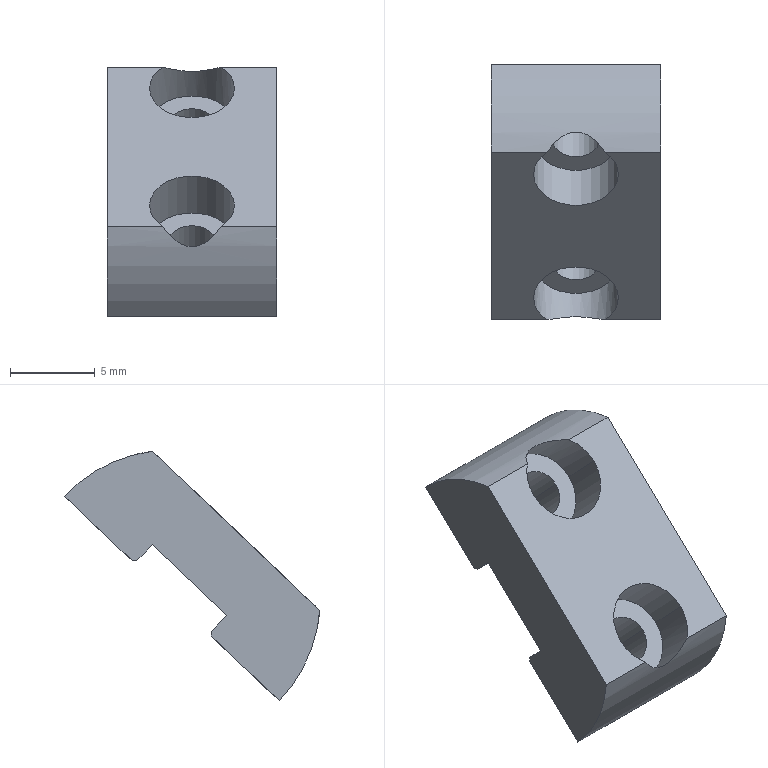Component | SolidWorks | JJDJR-3060-E-006-1 | 1 solid | 22 faces | box 10 x 15.06 x 14.71 mm | volume 656 mm3 | plane 12 | cylinder 10 | commonest cylinder face diameters 2.8 x4 5 x4 17.5 x2 | material 40Cr
build123d program:
from build123d import *

# Parameters (mm, degrees)
BOSS_EXTRUDE1_DEPTH                               = 5
M2_5_HEX_SOCKET_HEAD_CAP_SCREW_CBORE2_D           = 2.8
M2_5_HEX_SOCKET_HEAD_CAP_SCREW_CBORE2_CBORE_D     = 5
M2_5_HEX_SOCKET_HEAD_CAP_SCREW_CBORE2_CBORE_DEPTH = 6.5
CUT_EXTRUDE1_DEPTH                                = 16.91
CUT_EXTRUDE1_DEPTH_BACK                           = 16.91
CHAMFER1_SIZE                                     = 0.2


with BuildPart() as part:
    # Sketch1 → Boss-Extrude1 (new, symmetric)
    with BuildSketch(Plane.XY):
        with BuildLine():
            Line((-3.025, 0), (-8.75, 0))
            ThreePointArc((-8.75, 0), (0, 8.75), (8.75, 0))
            Line((8.75, 0), (3.025, 0))
            Line((3.025, 0), (3.025, 1.5))
            Line((3.025, 1.5), (-3.025, 1.5))
            Line((-3.025, 1.5), (-3.025, 0))
        make_face()
    extrude(amount=BOSS_EXTRUDE1_DEPTH, both=True)

    # M2.5 Hex Socket Head Cap Screw CBORE2 (through all)
    with Locations(Plane(origin=(0, 9, 0), x_dir=(1, 0, 0), z_dir=(0, 1, 0))):
        with Locations((5, 0), (-5, 0)):
            CounterBoreHole(M2_5_HEX_SOCKET_HEAD_CAP_SCREW_CBORE2_D / 2, M2_5_HEX_SOCKET_HEAD_CAP_SCREW_CBORE2_CBORE_D / 2, M2_5_HEX_SOCKET_HEAD_CAP_SCREW_CBORE2_CBORE_DEPTH)

    # Sketch4 → Cut-Extrude1 (cut, two sides: drawn at the far end of the back side and taken through both)
    with BuildSketch(Plane.XY.offset(5).offset(-CUT_EXTRUDE1_DEPTH_BACK)):
        Polygon((-57.338, 5.5), (-9.087, 5.5), (9.567, 5.5), (57.818, 5.5), (57.818, 102.002), (-57.338, 102.002), align=None)
    extrude(amount=CUT_EXTRUDE1_DEPTH + CUT_EXTRUDE1_DEPTH_BACK, mode=Mode.SUBTRACT)

    # Chamfer1
    chamfer1_edges = [part.edges().sort_by_distance(p)[0] for p in [
        (-3.025, 0, 0),
        (3.025, 0, 0),
    ]]
    chamfer(chamfer1_edges, length=CHAMFER1_SIZE)


solid = part.part

# Placed as in the assembly
solid = solid.moved(Location((-123.59, -29.263, -16.52), (133.57, 90, 0)))
STEP:
#1=COLOUR_RGB('',0.7922,0.8196,0.9333);
#2=FILL_AREA_STYLE_COLOUR('',#1);
#3=FILL_AREA_STYLE('',(#2));
#4=SURFACE_STYLE_FILL_AREA(#3);
#5=SURFACE_SIDE_STYLE('',(#4));
#6=SURFACE_STYLE_USAGE(.BOTH.,#5);
#7=PRESENTATION_STYLE_ASSIGNMENT((#6));
#8=CARTESIAN_POINT('',(-4.921,-1.009,-0.5147));
#9=VERTEX_POINT('',#8);
#10=CARTESIAN_POINT('',(-4.811,-1.009,-0.5147));
#11=VERTEX_POINT('',#10);
#12=CARTESIAN_POINT('',(-4.866,-1.009,-0.5147));
#13=DIRECTION('',(0.,-0.6892,0.7245));
#14=DIRECTION('',(1.,0.,0.));
#15=AXIS2_PLACEMENT_3D('',#12,#13,#14);
#16=CIRCLE('',#15,0.05512);
#17=EDGE_CURVE('',#9,#11,#16,.T.);
#18=ORIENTED_EDGE('',*,*,#17,.F.);
#19=CARTESIAN_POINT('',(-4.921,-1.077,-0.4434));
#20=VERTEX_POINT('',#19);
#21=CARTESIAN_POINT('',(-4.921,-1.254,-0.258));
#22=DIRECTION('',(0.,-0.6892,0.7245));
#23=VECTOR('',#22,39.37);
#24=LINE('',#21,#23);
#25=EDGE_CURVE('',#9,#20,#24,.T.);
#26=ORIENTED_EDGE('',*,*,#25,.T.);
#27=CARTESIAN_POINT('',(-4.811,-1.077,-0.4434));
#28=VERTEX_POINT('',#27);
#29=CARTESIAN_POINT('',(-4.866,-1.077,-0.4434));
#30=DIRECTION('',(0.,-0.6892,0.7245));
#31=DIRECTION('',(1.,0.,0.));
#32=AXIS2_PLACEMENT_3D('',#29,#30,#31);
#33=CIRCLE('',#32,0.05512);
#34=EDGE_CURVE('',#20,#28,#33,.T.);
#35=ORIENTED_EDGE('',*,*,#34,.T.);
#36=CARTESIAN_POINT('',(-4.811,-1.254,-0.258));
#37=DIRECTION('',(0.,-0.6892,0.7245));
#38=VECTOR('',#37,39.37);
#39=LINE('',#36,#38);
#40=EDGE_CURVE('',#11,#28,#39,.T.);
#41=ORIENTED_EDGE('',*,*,#40,.F.);
#42=EDGE_LOOP('',(#18,#26,#35,#41));
#43=FACE_OUTER_BOUND('',#42,.T.);
#44=CARTESIAN_POINT('',(-4.866,-1.254,-0.258));
#45=DIRECTION('',(0.,-0.6892,0.7245));
#46=DIRECTION('',(1.,0.,0.));
#47=AXIS2_PLACEMENT_3D('',#44,#45,#46);
#48=CYLINDRICAL_SURFACE('',#47,0.05512);
#49=ADVANCED_FACE('',(#43),#48,.F.);
#50=CARTESIAN_POINT('',(-4.921,-1.295,-0.7861));
#51=VERTEX_POINT('',#50);
#52=CARTESIAN_POINT('',(-4.811,-1.295,-0.7861));
#53=VERTEX_POINT('',#52);
#54=CARTESIAN_POINT('',(-4.866,-1.295,-0.7861));
#55=DIRECTION('',(0.,-0.6892,0.7245));
#56=DIRECTION('',(1.,0.,0.));
#57=AXIS2_PLACEMENT_3D('',#54,#55,#56);
#58=CIRCLE('',#57,0.05512);
#59=EDGE_CURVE('',#51,#53,#58,.T.);
#60=ORIENTED_EDGE('',*,*,#59,.F.);
#61=CARTESIAN_POINT('',(-4.921,-1.363,-0.7148));
#62=VERTEX_POINT('',#61);
#63=CARTESIAN_POINT('',(-4.921,-1.539,-0.5294));
#64=DIRECTION('',(0.,-0.6892,0.7245));
#65=VECTOR('',#64,39.37);
#66=LINE('',#63,#65);
#67=EDGE_CURVE('',#51,#62,#66,.T.);
#68=ORIENTED_EDGE('',*,*,#67,.T.);
#69=CARTESIAN_POINT('',(-4.811,-1.363,-0.7148));
#70=VERTEX_POINT('',#69);
#71=CARTESIAN_POINT('',(-4.866,-1.363,-0.7148));
#72=DIRECTION('',(0.,-0.6892,0.7245));
#73=DIRECTION('',(1.,0.,0.));
#74=AXIS2_PLACEMENT_3D('',#71,#72,#73);
#75=CIRCLE('',#74,0.05512);
#76=EDGE_CURVE('',#62,#70,#75,.T.);
#77=ORIENTED_EDGE('',*,*,#76,.T.);
#78=CARTESIAN_POINT('',(-4.811,-1.539,-0.5294));
#79=DIRECTION('',(0.,-0.6892,0.7245));
#80=VECTOR('',#79,39.37);
#81=LINE('',#78,#80);
#82=EDGE_CURVE('',#53,#70,#81,.T.);
#83=ORIENTED_EDGE('',*,*,#82,.F.);
#84=EDGE_LOOP('',(#60,#68,#77,#83));
#85=FACE_OUTER_BOUND('',#84,.T.);
#86=CARTESIAN_POINT('',(-4.866,-1.539,-0.5294));
#87=DIRECTION('',(0.,-0.6892,0.7245));
#88=DIRECTION('',(1.,0.,0.));
#89=AXIS2_PLACEMENT_3D('',#86,#87,#88);
#90=CYLINDRICAL_SURFACE('',#89,0.05512);
#91=ADVANCED_FACE('',(#85),#90,.F.);
#92=CARTESIAN_POINT('',(-4.964,-1.077,-0.4434));
#93=VERTEX_POINT('',#92);
#94=CARTESIAN_POINT('',(-4.767,-1.077,-0.4434));
#95=VERTEX_POINT('',#94);
#96=CARTESIAN_POINT('',(-4.866,-1.077,-0.4434));
#97=DIRECTION('',(0.,-0.6892,0.7245));
#98=DIRECTION('',(1.,0.,0.));
#99=AXIS2_PLACEMENT_3D('',#96,#97,#98);
#100=CIRCLE('',#99,0.09843);
#101=EDGE_CURVE('',#93,#95,#100,.T.);
#102=ORIENTED_EDGE('',*,*,#101,.F.);
#103=CARTESIAN_POINT('',(-4.964,-1.159,-0.3578));
#104=VERTEX_POINT('',#103);
#105=CARTESIAN_POINT('',(-4.964,-1.254,-0.258));
#106=DIRECTION('',(0.,-0.6892,0.7245));
#107=VECTOR('',#106,39.37);
#108=LINE('',#105,#107);
#109=EDGE_CURVE('',#93,#104,#108,.T.);
#110=ORIENTED_EDGE('',*,*,#109,.T.);
#111=CARTESIAN_POINT('',(-4.767,-1.159,-0.3578));
#112=VERTEX_POINT('',#111);
#113=CARTESIAN_POINT('',(-4.866,-1.159,-0.3578));
#114=DIRECTION('',(-0.,0.6892,-0.7245));
#115=DIRECTION('',(1.,0.,0.));
#116=AXIS2_PLACEMENT_3D('',#113,#114,#115);
#117=CIRCLE('',#116,0.09843);
#118=EDGE_CURVE('',#112,#104,#117,.T.);
#119=ORIENTED_EDGE('',*,*,#118,.F.);
#120=CARTESIAN_POINT('',(-4.767,-1.254,-0.258));
#121=DIRECTION('',(0.,-0.6892,0.7245));
#122=VECTOR('',#121,39.37);
#123=LINE('',#120,#122);
#124=EDGE_CURVE('',#95,#112,#123,.T.);
#125=ORIENTED_EDGE('',*,*,#124,.F.);
#126=EDGE_LOOP('',(#102,#110,#119,#125));
#127=FACE_OUTER_BOUND('',#126,.T.);
#128=CARTESIAN_POINT('',(-4.866,-1.254,-0.258));
#129=DIRECTION('',(0.,-0.6892,0.7245));
#130=DIRECTION('',(1.,0.,0.));
#131=AXIS2_PLACEMENT_3D('',#128,#129,#130);
#132=CYLINDRICAL_SURFACE('',#131,0.09843);
#133=ADVANCED_FACE('',(#127),#132,.F.);
#134=CARTESIAN_POINT('',(-4.964,-1.363,-0.7148));
#135=VERTEX_POINT('',#134);
#136=CARTESIAN_POINT('',(-4.767,-1.363,-0.7148));
#137=VERTEX_POINT('',#136);
#138=CARTESIAN_POINT('',(-4.866,-1.363,-0.7148));
#139=DIRECTION('',(0.,-0.6892,0.7245));
#140=DIRECTION('',(1.,0.,0.));
#141=AXIS2_PLACEMENT_3D('',#138,#139,#140);
#142=CIRCLE('',#141,0.09843);
#143=EDGE_CURVE('',#135,#137,#142,.T.);
#144=ORIENTED_EDGE('',*,*,#143,.F.);
#145=CARTESIAN_POINT('',(-4.964,-1.444,-0.6292));
#146=VERTEX_POINT('',#145);
#147=CARTESIAN_POINT('',(-4.964,-1.539,-0.5294));
#148=DIRECTION('',(0.,-0.6892,0.7245));
#149=VECTOR('',#148,39.37);
#150=LINE('',#147,#149);
#151=EDGE_CURVE('',#135,#146,#150,.T.);
#152=ORIENTED_EDGE('',*,*,#151,.T.);
#153=CARTESIAN_POINT('',(-4.934,-1.495,-0.6782));
#154=VERTEX_POINT('',#153);
#155=CARTESIAN_POINT('',(-4.866,-1.444,-0.6292));
#156=DIRECTION('',(-0.,0.6892,-0.7245));
#157=DIRECTION('',(1.,0.,0.));
#158=AXIS2_PLACEMENT_3D('',#155,#156,#157);
#159=CIRCLE('',#158,0.09843);
#160=EDGE_CURVE('',#154,#146,#159,.T.);
#161=ORIENTED_EDGE('',*,*,#160,.F.);
#162=CARTESIAN_POINT('',(-4.798,-1.495,-0.6782));
#163=VERTEX_POINT('',#162);
#164=CARTESIAN_POINT('',(-4.798,-1.495,-0.6782));
#165=CARTESIAN_POINT('',(-4.802,-1.495,-0.6842));
#166=CARTESIAN_POINT('',(-4.806,-1.494,-0.6899));
#167=CARTESIAN_POINT('',(-4.815,-1.493,-0.7007));
#168=CARTESIAN_POINT('',(-4.821,-1.492,-0.7057));
#169=CARTESIAN_POINT('',(-4.832,-1.491,-0.7146));
#170=CARTESIAN_POINT('',(-4.838,-1.49,-0.7184));
#171=CARTESIAN_POINT('',(-4.848,-1.489,-0.7225));
#172=CARTESIAN_POINT('',(-4.852,-1.489,-0.7235));
#173=CARTESIAN_POINT('',(-4.859,-1.488,-0.725));
#174=CARTESIAN_POINT('',(-4.862,-1.488,-0.7254));
#175=CARTESIAN_POINT('',(-4.873,-1.488,-0.7253));
#176=CARTESIAN_POINT('',(-4.88,-1.489,-0.7238));
#177=CARTESIAN_POINT('',(-4.894,-1.49,-0.7183));
#178=CARTESIAN_POINT('',(-4.9,-1.491,-0.7145));
#179=CARTESIAN_POINT('',(-4.917,-1.493,-0.7013));
#180=CARTESIAN_POINT('',(-4.926,-1.494,-0.6901));
#181=CARTESIAN_POINT('',(-4.934,-1.495,-0.6782));
#182=B_SPLINE_CURVE_WITH_KNOTS('',3,(#164,#165,#166,#167,#168,#169,#170,#171,#172,#173,#174,#175,#176,#177,#178,#179,#180,#181),.UNSPECIFIED.,.F.,.F.,(4,2,2,2,2,2,2,2,4),(0.002613,0.003158,0.003703,0.004248,0.004521,0.004793,0.005338,0.005883,0.006973),.UNSPECIFIED.);
#183=EDGE_CURVE('',#163,#154,#182,.T.);
#184=ORIENTED_EDGE('',*,*,#183,.F.);
#185=CARTESIAN_POINT('',(-4.767,-1.444,-0.6292));
#186=VERTEX_POINT('',#185);
#187=CARTESIAN_POINT('',(-4.866,-1.444,-0.6292));
#188=DIRECTION('',(-0.,0.6892,-0.7245));
#189=DIRECTION('',(1.,0.,0.));
#190=AXIS2_PLACEMENT_3D('',#187,#188,#189);
#191=CIRCLE('',#190,0.09843);
#192=EDGE_CURVE('',#186,#163,#191,.T.);
#193=ORIENTED_EDGE('',*,*,#192,.F.);
#194=CARTESIAN_POINT('',(-4.767,-1.539,-0.5294));
#195=DIRECTION('',(0.,-0.6892,0.7245));
#196=VECTOR('',#195,39.37);
#197=LINE('',#194,#196);
#198=EDGE_CURVE('',#137,#186,#197,.T.);
#199=ORIENTED_EDGE('',*,*,#198,.F.);
#200=EDGE_LOOP('',(#144,#152,#161,#184,#193,#199));
#201=FACE_OUTER_BOUND('',#200,.T.);
#202=CARTESIAN_POINT('',(-4.866,-1.539,-0.5294));
#203=DIRECTION('',(0.,-0.6892,0.7245));
#204=DIRECTION('',(1.,0.,0.));
#205=AXIS2_PLACEMENT_3D('',#202,#203,#204);
#206=CYLINDRICAL_SURFACE('',#205,0.09843);
#207=ADVANCED_FACE('',(#201),#206,.F.);
#208=CARTESIAN_POINT('',(-4.669,-1.107,-0.3088));
#209=VERTEX_POINT('',#208);
#210=CARTESIAN_POINT('',(-4.798,-1.107,-0.3088));
#211=VERTEX_POINT('',#210);
#212=CARTESIAN_POINT('',(-4.669,-1.107,-0.3088));
#213=DIRECTION('',(-1.,-0.,0.));
#214=VECTOR('',#213,39.37);
#215=LINE('',#212,#214);
#216=EDGE_CURVE('',#209,#211,#215,.T.);
#217=ORIENTED_EDGE('',*,*,#216,.F.);
#218=CARTESIAN_POINT('',(-4.669,-0.9025,-0.413));
#219=VERTEX_POINT('',#218);
#220=CARTESIAN_POINT('',(-4.669,-1.152,-0.6504));
#221=DIRECTION('',(1.,0.,-0.));
#222=DIRECTION('',(0.,0.7245,0.6892));
#223=AXIS2_PLACEMENT_3D('',#220,#221,#222);
#224=CIRCLE('',#223,0.3445);
#225=EDGE_CURVE('',#219,#209,#224,.T.);
#226=ORIENTED_EDGE('',*,*,#225,.F.);
#227=CARTESIAN_POINT('',(-5.063,-0.9025,-0.413));
#228=VERTEX_POINT('',#227);
#229=CARTESIAN_POINT('',(-4.669,-0.9025,-0.413));
#230=DIRECTION('',(-1.,-0.,0.));
#231=VECTOR('',#230,39.37);
#232=LINE('',#229,#231);
#233=EDGE_CURVE('',#219,#228,#232,.T.);
#234=ORIENTED_EDGE('',*,*,#233,.T.);
#235=CARTESIAN_POINT('',(-5.063,-1.107,-0.3088));
#236=VERTEX_POINT('',#235);
#237=CARTESIAN_POINT('',(-5.063,-1.152,-0.6504));
#238=DIRECTION('',(1.,0.,-0.));
#239=DIRECTION('',(0.,0.7245,0.6892));
#240=AXIS2_PLACEMENT_3D('',#237,#238,#239);
#241=CIRCLE('',#240,0.3445);
#242=EDGE_CURVE('',#228,#236,#241,.T.);
#243=ORIENTED_EDGE('',*,*,#242,.T.);
#244=CARTESIAN_POINT('',(-4.934,-1.107,-0.3088));
#245=VERTEX_POINT('',#244);
#246=CARTESIAN_POINT('',(-4.669,-1.107,-0.3088));
#247=DIRECTION('',(-1.,-0.,0.));
#248=VECTOR('',#247,39.37);
#249=LINE('',#246,#248);
#250=EDGE_CURVE('',#245,#236,#249,.T.);
#251=ORIENTED_EDGE('',*,*,#250,.F.);
#252=CARTESIAN_POINT('',(-4.934,-1.107,-0.3088));
#253=CARTESIAN_POINT('',(-4.93,-1.101,-0.3096));
#254=CARTESIAN_POINT('',(-4.926,-1.096,-0.3105));
#255=CARTESIAN_POINT('',(-4.916,-1.085,-0.3125));
#256=CARTESIAN_POINT('',(-4.911,-1.08,-0.3135));
#257=CARTESIAN_POINT('',(-4.9,-1.071,-0.3155));
#258=CARTESIAN_POINT('',(-4.893,-1.067,-0.3165));
#259=CARTESIAN_POINT('',(-4.88,-1.062,-0.3179));
#260=CARTESIAN_POINT('',(-4.873,-1.06,-0.3183));
#261=CARTESIAN_POINT('',(-4.858,-1.06,-0.3183));
#262=CARTESIAN_POINT('',(-4.851,-1.062,-0.3179));
#263=CARTESIAN_POINT('',(-4.838,-1.067,-0.3165));
#264=CARTESIAN_POINT('',(-4.832,-1.071,-0.3155));
#265=CARTESIAN_POINT('',(-4.82,-1.08,-0.3135));
#266=CARTESIAN_POINT('',(-4.815,-1.085,-0.3125));
#267=CARTESIAN_POINT('',(-4.806,-1.096,-0.3105));
#268=CARTESIAN_POINT('',(-4.802,-1.101,-0.3096));
#269=CARTESIAN_POINT('',(-4.798,-1.107,-0.3088));
#270=B_SPLINE_CURVE_WITH_KNOTS('',3,(#252,#253,#254,#255,#256,#257,#258,#259,#260,#261,#262,#263,#264,#265,#266,#267,#268,#269),.UNSPECIFIED.,.F.,.F.,(4,2,2,2,2,2,2,2,4),(0.01092,0.01147,0.01201,0.01255,0.0131,0.01364,0.01419,0.01473,0.01528),.UNSPECIFIED.);
#271=EDGE_CURVE('',#245,#211,#270,.T.);
#272=ORIENTED_EDGE('',*,*,#271,.T.);
#273=EDGE_LOOP('',(#217,#226,#234,#243,#251,#272));
#274=FACE_OUTER_BOUND('',#273,.T.);
#275=CARTESIAN_POINT('',(-4.669,-1.152,-0.6504));
#276=DIRECTION('',(-1.,-0.,0.));
#277=DIRECTION('',(0.,-0.7245,-0.6892));
#278=AXIS2_PLACEMENT_3D('',#275,#276,#277);
#279=CYLINDRICAL_SURFACE('',#278,0.3445);
#280=ADVANCED_FACE('',(#274),#279,.T.);
#281=CARTESIAN_POINT('',(-5.063,-1.495,-0.6782));
#282=VERTEX_POINT('',#281);
#283=CARTESIAN_POINT('',(-4.669,-1.495,-0.6782));
#284=DIRECTION('',(1.,0.,-0.));
#285=VECTOR('',#284,39.37);
#286=LINE('',#283,#285);
#287=EDGE_CURVE('',#282,#154,#286,.T.);
#288=ORIENTED_EDGE('',*,*,#287,.F.);
#289=CARTESIAN_POINT('',(-5.063,-1.402,-0.8878));
#290=VERTEX_POINT('',#289);
#291=CARTESIAN_POINT('',(-5.063,-1.152,-0.6504));
#292=DIRECTION('',(1.,0.,-0.));
#293=DIRECTION('',(0.,0.7245,0.6892));
#294=AXIS2_PLACEMENT_3D('',#291,#292,#293);
#295=CIRCLE('',#294,0.3445);
#296=EDGE_CURVE('',#282,#290,#295,.T.);
#297=ORIENTED_EDGE('',*,*,#296,.T.);
#298=CARTESIAN_POINT('',(-4.669,-1.402,-0.8878));
#299=VERTEX_POINT('',#298);
#300=CARTESIAN_POINT('',(-4.669,-1.402,-0.8878));
#301=DIRECTION('',(-1.,-0.,0.));
#302=VECTOR('',#301,39.37);
#303=LINE('',#300,#302);
#304=EDGE_CURVE('',#299,#290,#303,.T.);
#305=ORIENTED_EDGE('',*,*,#304,.F.);
#306=CARTESIAN_POINT('',(-4.669,-1.495,-0.6782));
#307=VERTEX_POINT('',#306);
#308=CARTESIAN_POINT('',(-4.669,-1.152,-0.6504));
#309=DIRECTION('',(1.,0.,-0.));
#310=DIRECTION('',(0.,0.7245,0.6892));
#311=AXIS2_PLACEMENT_3D('',#308,#309,#310);
#312=CIRCLE('',#311,0.3445);
#313=EDGE_CURVE('',#307,#299,#312,.T.);
#314=ORIENTED_EDGE('',*,*,#313,.F.);
#315=CARTESIAN_POINT('',(-4.669,-1.495,-0.6782));
#316=DIRECTION('',(1.,0.,-0.));
#317=VECTOR('',#316,39.37);
#318=LINE('',#315,#317);
#319=EDGE_CURVE('',#163,#307,#318,.T.);
#320=ORIENTED_EDGE('',*,*,#319,.F.);
#321=ORIENTED_EDGE('',*,*,#183,.T.);
#322=EDGE_LOOP('',(#288,#297,#305,#314,#320,#321));
#323=FACE_OUTER_BOUND('',#322,.T.);
#324=CARTESIAN_POINT('',(-4.669,-1.152,-0.6504));
#325=DIRECTION('',(-1.,-0.,0.));
#326=DIRECTION('',(0.,-0.7245,-0.6892));
#327=AXIS2_PLACEMENT_3D('',#324,#325,#326);
#328=CYLINDRICAL_SURFACE('',#327,0.3445);
#329=ADVANCED_FACE('',(#323),#328,.T.);
#330=CARTESIAN_POINT('',(-4.669,-1.106,-0.5255));
#331=VERTEX_POINT('',#330);
#332=CARTESIAN_POINT('',(-4.669,-1.071,-0.5626));
#333=VERTEX_POINT('',#332);
#334=CARTESIAN_POINT('',(-4.669,-1.066,-0.5683));
#335=DIRECTION('',(-0.,0.6892,-0.7245));
#336=VECTOR('',#335,39.37);
#337=LINE('',#334,#336);
#338=EDGE_CURVE('',#331,#333,#337,.T.);
#339=ORIENTED_EDGE('',*,*,#338,.T.);
#340=CARTESIAN_POINT('',(-4.669,-1.06,-0.5629));
#341=VERTEX_POINT('',#340);
#342=CARTESIAN_POINT('',(-4.669,-1.15,-0.5606));
#343=DIRECTION('',(-0.,0.9997,-0.02495));
#344=VECTOR('',#343,39.37);
#345=LINE('',#342,#344);
#346=EDGE_CURVE('',#333,#341,#345,.T.);
#347=ORIENTED_EDGE('',*,*,#346,.T.);
#348=CARTESIAN_POINT('',(-4.669,-1.066,-0.5683));
#349=DIRECTION('',(0.,0.7245,0.6892));
#350=VECTOR('',#349,39.37);
#351=LINE('',#348,#350);
#352=EDGE_CURVE('',#341,#219,#351,.T.);
#353=ORIENTED_EDGE('',*,*,#352,.T.);
#354=ORIENTED_EDGE('',*,*,#225,.T.);
#355=CARTESIAN_POINT('',(-4.669,-1.301,-0.4935));
#356=DIRECTION('',(-0.,-0.7245,-0.6892));
#357=VECTOR('',#356,39.37);
#358=LINE('',#355,#357);
#359=EDGE_CURVE('',#209,#307,#358,.T.);
#360=ORIENTED_EDGE('',*,*,#359,.T.);
#361=ORIENTED_EDGE('',*,*,#313,.T.);
#362=CARTESIAN_POINT('',(-4.669,-1.244,-0.7379));
#363=VERTEX_POINT('',#362);
#364=CARTESIAN_POINT('',(-4.669,-1.238,-0.7325));
#365=DIRECTION('',(0.,0.7245,0.6892));
#366=VECTOR('',#365,39.37);
#367=LINE('',#364,#366);
#368=EDGE_CURVE('',#299,#363,#367,.T.);
#369=ORIENTED_EDGE('',*,*,#368,.T.);
#370=CARTESIAN_POINT('',(-4.669,-1.244,-0.7268));
#371=VERTEX_POINT('',#370);
#372=CARTESIAN_POINT('',(-4.669,-1.242,-0.6482));
#373=DIRECTION('',(0.,0.02495,0.9997));
#374=VECTOR('',#373,39.37);
#375=LINE('',#372,#374);
#376=EDGE_CURVE('',#363,#371,#375,.T.);
#377=ORIENTED_EDGE('',*,*,#376,.T.);
#378=CARTESIAN_POINT('',(-4.669,-1.279,-0.6897));
#379=VERTEX_POINT('',#378);
#380=CARTESIAN_POINT('',(-4.669,-1.238,-0.7325));
#381=DIRECTION('',(0.,-0.6892,0.7245));
#382=VECTOR('',#381,39.37);
#383=LINE('',#380,#382);
#384=EDGE_CURVE('',#371,#379,#383,.T.);
#385=ORIENTED_EDGE('',*,*,#384,.T.);
#386=CARTESIAN_POINT('',(-4.669,-1.279,-0.6897));
#387=DIRECTION('',(0.,0.7245,0.6892));
#388=VECTOR('',#387,39.37);
#389=LINE('',#386,#388);
#390=EDGE_CURVE('',#379,#331,#389,.T.);
#391=ORIENTED_EDGE('',*,*,#390,.T.);
#392=EDGE_LOOP('',(#339,#347,#353,#354,#360,#361,#369,#377,#385,#391));
#393=FACE_OUTER_BOUND('',#392,.T.);
#394=CARTESIAN_POINT('',(-4.669,-1.152,-0.6504));
#395=DIRECTION('',(1.,0.,-0.));
#396=DIRECTION('',(0.,0.7245,0.6892));
#397=AXIS2_PLACEMENT_3D('',#394,#395,#396);
#398=PLANE('',#397);
#399=ADVANCED_FACE('',(#393),#398,.T.);
#400=CARTESIAN_POINT('',(-5.063,-1.06,-0.5629));
#401=VERTEX_POINT('',#400);
#402=CARTESIAN_POINT('',(-5.063,-1.066,-0.5683));
#403=DIRECTION('',(0.,0.7245,0.6892));
#404=VECTOR('',#403,39.37);
#405=LINE('',#402,#404);
#406=EDGE_CURVE('',#401,#228,#405,.T.);
#407=ORIENTED_EDGE('',*,*,#406,.F.);
#408=CARTESIAN_POINT('',(-5.063,-1.071,-0.5626));
#409=VERTEX_POINT('',#408);
#410=CARTESIAN_POINT('',(-5.063,-1.06,-0.5629));
#411=DIRECTION('',(0.,-0.9997,0.02495));
#412=VECTOR('',#411,39.37);
#413=LINE('',#410,#412);
#414=EDGE_CURVE('',#401,#409,#413,.T.);
#415=ORIENTED_EDGE('',*,*,#414,.T.);
#416=CARTESIAN_POINT('',(-5.063,-1.106,-0.5255));
#417=VERTEX_POINT('',#416);
#418=CARTESIAN_POINT('',(-5.063,-1.066,-0.5683));
#419=DIRECTION('',(-0.,0.6892,-0.7245));
#420=VECTOR('',#419,39.37);
#421=LINE('',#418,#420);
#422=EDGE_CURVE('',#417,#409,#421,.T.);
#423=ORIENTED_EDGE('',*,*,#422,.F.);
#424=CARTESIAN_POINT('',(-5.063,-1.279,-0.6897));
#425=VERTEX_POINT('',#424);
#426=CARTESIAN_POINT('',(-5.063,-1.279,-0.6897));
#427=DIRECTION('',(0.,0.7245,0.6892));
#428=VECTOR('',#427,39.37);
#429=LINE('',#426,#428);
#430=EDGE_CURVE('',#425,#417,#429,.T.);
#431=ORIENTED_EDGE('',*,*,#430,.F.);
#432=CARTESIAN_POINT('',(-5.063,-1.244,-0.7268));
#433=VERTEX_POINT('',#432);
#434=CARTESIAN_POINT('',(-5.063,-1.238,-0.7325));
#435=DIRECTION('',(0.,-0.6892,0.7245));
#436=VECTOR('',#435,39.37);
#437=LINE('',#434,#436);
#438=EDGE_CURVE('',#433,#425,#437,.T.);
#439=ORIENTED_EDGE('',*,*,#438,.F.);
#440=CARTESIAN_POINT('',(-5.063,-1.244,-0.7379));
#441=VERTEX_POINT('',#440);
#442=CARTESIAN_POINT('',(-5.063,-1.244,-0.7268));
#443=DIRECTION('',(-0.,-0.02495,-0.9997));
#444=VECTOR('',#443,39.37);
#445=LINE('',#442,#444);
#446=EDGE_CURVE('',#433,#441,#445,.T.);
#447=ORIENTED_EDGE('',*,*,#446,.T.);
#448=CARTESIAN_POINT('',(-5.063,-1.238,-0.7325));
#449=DIRECTION('',(0.,0.7245,0.6892));
#450=VECTOR('',#449,39.37);
#451=LINE('',#448,#450);
#452=EDGE_CURVE('',#290,#441,#451,.T.);
#453=ORIENTED_EDGE('',*,*,#452,.F.);
#454=ORIENTED_EDGE('',*,*,#296,.F.);
#455=CARTESIAN_POINT('',(-5.063,-1.301,-0.4935));
#456=DIRECTION('',(-0.,-0.7245,-0.6892));
#457=VECTOR('',#456,39.37);
#458=LINE('',#455,#457);
#459=EDGE_CURVE('',#236,#282,#458,.T.);
#460=ORIENTED_EDGE('',*,*,#459,.F.);
#461=ORIENTED_EDGE('',*,*,#242,.F.);
#462=EDGE_LOOP('',(#407,#415,#423,#431,#439,#447,#453,#454,#460,#461));
#463=FACE_OUTER_BOUND('',#462,.T.);
#464=CARTESIAN_POINT('',(-5.063,-1.152,-0.6504));
#465=DIRECTION('',(1.,0.,-0.));
#466=DIRECTION('',(0.,0.7245,0.6892));
#467=AXIS2_PLACEMENT_3D('',#464,#465,#466);
#468=PLANE('',#467);
#469=ADVANCED_FACE('',(#463),#468,.F.);
#470=ORIENTED_EDGE('',*,*,#151,.F.);
#471=CARTESIAN_POINT('',(-4.866,-1.363,-0.7148));
#472=DIRECTION('',(0.,-0.6892,0.7245));
#473=DIRECTION('',(1.,0.,0.));
#474=AXIS2_PLACEMENT_3D('',#471,#472,#473);
#475=CIRCLE('',#474,0.09843);
#476=EDGE_CURVE('',#137,#135,#475,.T.);
#477=ORIENTED_EDGE('',*,*,#476,.F.);
#478=ORIENTED_EDGE('',*,*,#198,.T.);
#479=CARTESIAN_POINT('',(-4.866,-1.444,-0.6292));
#480=DIRECTION('',(-0.,0.6892,-0.7245));
#481=DIRECTION('',(1.,0.,0.));
#482=AXIS2_PLACEMENT_3D('',#479,#480,#481);
#483=CIRCLE('',#482,0.09843);
#484=EDGE_CURVE('',#146,#186,#483,.T.);
#485=ORIENTED_EDGE('',*,*,#484,.F.);
#486=EDGE_LOOP('',(#470,#477,#478,#485));
#487=FACE_OUTER_BOUND('',#486,.T.);
#488=CARTESIAN_POINT('',(-4.866,-1.539,-0.5294));
#489=DIRECTION('',(0.,-0.6892,0.7245));
#490=DIRECTION('',(1.,0.,0.));
#491=AXIS2_PLACEMENT_3D('',#488,#489,#490);
#492=CYLINDRICAL_SURFACE('',#491,0.09843);
#493=ADVANCED_FACE('',(#487),#492,.F.);
#494=ORIENTED_EDGE('',*,*,#109,.F.);
#495=CARTESIAN_POINT('',(-4.866,-1.077,-0.4434));
#496=DIRECTION('',(0.,-0.6892,0.7245));
#497=DIRECTION('',(1.,0.,0.));
#498=AXIS2_PLACEMENT_3D('',#495,#496,#497);
#499=CIRCLE('',#498,0.09843);
#500=EDGE_CURVE('',#95,#93,#499,.T.);
#501=ORIENTED_EDGE('',*,*,#500,.F.);
#502=ORIENTED_EDGE('',*,*,#124,.T.);
#503=CARTESIAN_POINT('',(-4.866,-1.159,-0.3578));
#504=DIRECTION('',(-0.,0.6892,-0.7245));
#505=DIRECTION('',(1.,0.,0.));
#506=AXIS2_PLACEMENT_3D('',#503,#504,#505);
#507=CIRCLE('',#506,0.09843);
#508=EDGE_CURVE('',#211,#112,#507,.T.);
#509=ORIENTED_EDGE('',*,*,#508,.F.);
#510=ORIENTED_EDGE('',*,*,#271,.F.);
#511=CARTESIAN_POINT('',(-4.866,-1.159,-0.3578));
#512=DIRECTION('',(-0.,0.6892,-0.7245));
#513=DIRECTION('',(1.,0.,0.));
#514=AXIS2_PLACEMENT_3D('',#511,#512,#513);
#515=CIRCLE('',#514,0.09843);
#516=EDGE_CURVE('',#104,#245,#515,.T.);
#517=ORIENTED_EDGE('',*,*,#516,.F.);
#518=EDGE_LOOP('',(#494,#501,#502,#509,#510,#517));
#519=FACE_OUTER_BOUND('',#518,.T.);
#520=CARTESIAN_POINT('',(-4.866,-1.254,-0.258));
#521=DIRECTION('',(0.,-0.6892,0.7245));
#522=DIRECTION('',(1.,0.,0.));
#523=AXIS2_PLACEMENT_3D('',#520,#521,#522);
#524=CYLINDRICAL_SURFACE('',#523,0.09843);
#525=ADVANCED_FACE('',(#519),#524,.F.);
#526=ORIENTED_EDGE('',*,*,#422,.T.);
#527=CARTESIAN_POINT('',(-4.669,-1.071,-0.5626));
#528=DIRECTION('',(1.,0.,-0.));
#529=VECTOR('',#528,39.37);
#530=LINE('',#527,#529);
#531=EDGE_CURVE('',#409,#333,#530,.T.);
#532=ORIENTED_EDGE('',*,*,#531,.T.);
#533=ORIENTED_EDGE('',*,*,#338,.F.);
#534=CARTESIAN_POINT('',(-4.669,-1.106,-0.5255));
#535=DIRECTION('',(-1.,-0.,0.));
#536=VECTOR('',#535,39.37);
#537=LINE('',#534,#536);
#538=EDGE_CURVE('',#331,#417,#537,.T.);
#539=ORIENTED_EDGE('',*,*,#538,.T.);
#540=EDGE_LOOP('',(#526,#532,#533,#539));
#541=FACE_OUTER_BOUND('',#540,.T.);
#542=CARTESIAN_POINT('',(-4.669,-1.066,-0.5683));
#543=DIRECTION('',(0.,0.7245,0.6892));
#544=DIRECTION('',(-1.,-0.,0.));
#545=AXIS2_PLACEMENT_3D('',#542,#543,#544);
#546=PLANE('',#545);
#547=ADVANCED_FACE('',(#541),#546,.F.);
#548=CARTESIAN_POINT('',(-4.866,-1.009,-0.5147));
#549=DIRECTION('',(0.,-0.6892,0.7245));
#550=DIRECTION('',(1.,0.,0.));
#551=AXIS2_PLACEMENT_3D('',#548,#549,#550);
#552=CIRCLE('',#551,0.05512);
#553=EDGE_CURVE('',#11,#9,#552,.T.);
#554=ORIENTED_EDGE('',*,*,#553,.T.);
#555=ORIENTED_EDGE('',*,*,#17,.T.);
#556=EDGE_LOOP('',(#554,#555));
#557=FACE_BOUND('',#556,.T.);
#558=ORIENTED_EDGE('',*,*,#352,.F.);
#559=CARTESIAN_POINT('',(-4.669,-1.06,-0.5629));
#560=DIRECTION('',(-1.,-0.,0.));
#561=VECTOR('',#560,39.37);
#562=LINE('',#559,#561);
#563=EDGE_CURVE('',#341,#401,#562,.T.);
#564=ORIENTED_EDGE('',*,*,#563,.T.);
#565=ORIENTED_EDGE('',*,*,#406,.T.);
#566=ORIENTED_EDGE('',*,*,#233,.F.);
#567=EDGE_LOOP('',(#558,#564,#565,#566));
#568=FACE_OUTER_BOUND('',#567,.T.);
#569=CARTESIAN_POINT('',(-4.669,-1.066,-0.5683));
#570=DIRECTION('',(0.,-0.6892,0.7245));
#571=DIRECTION('',(-0.,-0.7245,-0.6892));
#572=AXIS2_PLACEMENT_3D('',#569,#570,#571);
#573=PLANE('',#572);
#574=ADVANCED_FACE('',(#557,#568),#573,.F.);
#575=CARTESIAN_POINT('',(-4.866,-1.295,-0.7861));
#576=DIRECTION('',(0.,-0.6892,0.7245));
#577=DIRECTION('',(1.,0.,0.));
#578=AXIS2_PLACEMENT_3D('',#575,#576,#577);
#579=CIRCLE('',#578,0.05512);
#580=EDGE_CURVE('',#53,#51,#579,.T.);
#581=ORIENTED_EDGE('',*,*,#580,.T.);
#582=ORIENTED_EDGE('',*,*,#59,.T.);
#583=EDGE_LOOP('',(#581,#582));
#584=FACE_BOUND('',#583,.T.);
#585=ORIENTED_EDGE('',*,*,#452,.T.);
#586=CARTESIAN_POINT('',(-4.669,-1.244,-0.7379));
#587=DIRECTION('',(1.,0.,-0.));
#588=VECTOR('',#587,39.37);
#589=LINE('',#586,#588);
#590=EDGE_CURVE('',#441,#363,#589,.T.);
#591=ORIENTED_EDGE('',*,*,#590,.T.);
#592=ORIENTED_EDGE('',*,*,#368,.F.);
#593=ORIENTED_EDGE('',*,*,#304,.T.);
#594=EDGE_LOOP('',(#585,#591,#592,#593));
#595=FACE_OUTER_BOUND('',#594,.T.);
#596=CARTESIAN_POINT('',(-4.669,-1.238,-0.7325));
#597=DIRECTION('',(0.,-0.6892,0.7245));
#598=DIRECTION('',(-0.,-0.7245,-0.6892));
#599=AXIS2_PLACEMENT_3D('',#596,#597,#598);
#600=PLANE('',#599);
#601=ADVANCED_FACE('',(#584,#595),#600,.F.);
#602=ORIENTED_EDGE('',*,*,#384,.F.);
#603=CARTESIAN_POINT('',(-4.669,-1.244,-0.7268));
#604=DIRECTION('',(-1.,-0.,0.));
#605=VECTOR('',#604,39.37);
#606=LINE('',#603,#605);
#607=EDGE_CURVE('',#371,#433,#606,.T.);
#608=ORIENTED_EDGE('',*,*,#607,.T.);
#609=ORIENTED_EDGE('',*,*,#438,.T.);
#610=CARTESIAN_POINT('',(-4.669,-1.279,-0.6897));
#611=DIRECTION('',(-1.,-0.,0.));
#612=VECTOR('',#611,39.37);
#613=LINE('',#610,#612);
#614=EDGE_CURVE('',#379,#425,#613,.T.);
#615=ORIENTED_EDGE('',*,*,#614,.F.);
#616=EDGE_LOOP('',(#602,#608,#609,#615));
#617=FACE_OUTER_BOUND('',#616,.T.);
#618=CARTESIAN_POINT('',(-4.669,-1.238,-0.7325));
#619=DIRECTION('',(-0.,-0.7245,-0.6892));
#620=DIRECTION('',(1.,0.,-0.));
#621=AXIS2_PLACEMENT_3D('',#618,#619,#620);
#622=PLANE('',#621);
#623=ADVANCED_FACE('',(#617),#622,.F.);
#624=ORIENTED_EDGE('',*,*,#430,.T.);
#625=ORIENTED_EDGE('',*,*,#538,.F.);
#626=ORIENTED_EDGE('',*,*,#390,.F.);
#627=ORIENTED_EDGE('',*,*,#614,.T.);
#628=EDGE_LOOP('',(#624,#625,#626,#627));
#629=FACE_OUTER_BOUND('',#628,.T.);
#630=CARTESIAN_POINT('',(-4.669,-1.279,-0.6897));
#631=DIRECTION('',(0.,-0.6892,0.7245));
#632=DIRECTION('',(1.,0.,-0.));
#633=AXIS2_PLACEMENT_3D('',#630,#631,#632);
#634=PLANE('',#633);
#635=ADVANCED_FACE('',(#629),#634,.F.);
#636=ORIENTED_EDGE('',*,*,#67,.F.);
#637=ORIENTED_EDGE('',*,*,#580,.F.);
#638=ORIENTED_EDGE('',*,*,#82,.T.);
#639=CARTESIAN_POINT('',(-4.866,-1.363,-0.7148));
#640=DIRECTION('',(0.,-0.6892,0.7245));
#641=DIRECTION('',(1.,0.,0.));
#642=AXIS2_PLACEMENT_3D('',#639,#640,#641);
#643=CIRCLE('',#642,0.05512);
#644=EDGE_CURVE('',#70,#62,#643,.T.);
#645=ORIENTED_EDGE('',*,*,#644,.T.);
#646=EDGE_LOOP('',(#636,#637,#638,#645));
#647=FACE_OUTER_BOUND('',#646,.T.);
#648=CARTESIAN_POINT('',(-4.866,-1.539,-0.5294));
#649=DIRECTION('',(0.,-0.6892,0.7245));
#650=DIRECTION('',(1.,0.,0.));
#651=AXIS2_PLACEMENT_3D('',#648,#649,#650);
#652=CYLINDRICAL_SURFACE('',#651,0.05512);
#653=ADVANCED_FACE('',(#647),#652,.F.);
#654=ORIENTED_EDGE('',*,*,#644,.F.);
#655=ORIENTED_EDGE('',*,*,#76,.F.);
#656=EDGE_LOOP('',(#654,#655));
#657=FACE_BOUND('',#656,.T.);
#658=ORIENTED_EDGE('',*,*,#476,.T.);
#659=ORIENTED_EDGE('',*,*,#143,.T.);
#660=EDGE_LOOP('',(#658,#659));
#661=FACE_OUTER_BOUND('',#660,.T.);
#662=CARTESIAN_POINT('',(-4.866,-1.323,-0.6768));
#663=DIRECTION('',(-0.,0.6892,-0.7245));
#664=DIRECTION('',(-1.,-0.,0.));
#665=AXIS2_PLACEMENT_3D('',#662,#663,#664);
#666=PLANE('',#665);
#667=ADVANCED_FACE('',(#657,#661),#666,.F.);
#668=ORIENTED_EDGE('',*,*,#25,.F.);
#669=ORIENTED_EDGE('',*,*,#553,.F.);
#670=ORIENTED_EDGE('',*,*,#40,.T.);
#671=CARTESIAN_POINT('',(-4.866,-1.077,-0.4434));
#672=DIRECTION('',(0.,-0.6892,0.7245));
#673=DIRECTION('',(1.,0.,0.));
#674=AXIS2_PLACEMENT_3D('',#671,#672,#673);
#675=CIRCLE('',#674,0.05512);
#676=EDGE_CURVE('',#28,#20,#675,.T.);
#677=ORIENTED_EDGE('',*,*,#676,.T.);
#678=EDGE_LOOP('',(#668,#669,#670,#677));
#679=FACE_OUTER_BOUND('',#678,.T.);
#680=CARTESIAN_POINT('',(-4.866,-1.254,-0.258));
#681=DIRECTION('',(0.,-0.6892,0.7245));
#682=DIRECTION('',(1.,0.,0.));
#683=AXIS2_PLACEMENT_3D('',#680,#681,#682);
#684=CYLINDRICAL_SURFACE('',#683,0.05512);
#685=ADVANCED_FACE('',(#679),#684,.F.);
#686=ORIENTED_EDGE('',*,*,#676,.F.);
#687=ORIENTED_EDGE('',*,*,#34,.F.);
#688=EDGE_LOOP('',(#686,#687));
#689=FACE_BOUND('',#688,.T.);
#690=ORIENTED_EDGE('',*,*,#500,.T.);
#691=ORIENTED_EDGE('',*,*,#101,.T.);
#692=EDGE_LOOP('',(#690,#691));
#693=FACE_OUTER_BOUND('',#692,.T.);
#694=CARTESIAN_POINT('',(-4.866,-1.037,-0.4054));
#695=DIRECTION('',(-0.,0.6892,-0.7245));
#696=DIRECTION('',(-1.,-0.,0.));
#697=AXIS2_PLACEMENT_3D('',#694,#695,#696);
#698=PLANE('',#697);
#699=ADVANCED_FACE('',(#689,#693),#698,.F.);
#700=ORIENTED_EDGE('',*,*,#287,.T.);
#701=ORIENTED_EDGE('',*,*,#160,.T.);
#702=ORIENTED_EDGE('',*,*,#484,.T.);
#703=ORIENTED_EDGE('',*,*,#192,.T.);
#704=ORIENTED_EDGE('',*,*,#319,.T.);
#705=ORIENTED_EDGE('',*,*,#359,.F.);
#706=ORIENTED_EDGE('',*,*,#216,.T.);
#707=ORIENTED_EDGE('',*,*,#508,.T.);
#708=ORIENTED_EDGE('',*,*,#118,.T.);
#709=ORIENTED_EDGE('',*,*,#516,.T.);
#710=ORIENTED_EDGE('',*,*,#250,.T.);
#711=ORIENTED_EDGE('',*,*,#459,.T.);
#712=EDGE_LOOP('',(#700,#701,#702,#703,#704,#705,#706,#707,#708,#709,#710,#711));
#713=FACE_OUTER_BOUND('',#712,.T.);
#714=CARTESIAN_POINT('',(-3.095,-1.561,-0.7401));
#715=DIRECTION('',(0.,-0.6892,0.7245));
#716=DIRECTION('',(1.,0.,-0.));
#717=AXIS2_PLACEMENT_3D('',#714,#715,#716);
#718=PLANE('',#717);
#719=ADVANCED_FACE('',(#713),#718,.T.);
#720=ORIENTED_EDGE('',*,*,#346,.F.);
#721=ORIENTED_EDGE('',*,*,#531,.F.);
#722=ORIENTED_EDGE('',*,*,#414,.F.);
#723=ORIENTED_EDGE('',*,*,#563,.F.);
#724=EDGE_LOOP('',(#720,#721,#722,#723));
#725=FACE_OUTER_BOUND('',#724,.T.);
#726=CARTESIAN_POINT('',(-4.669,-1.06,-0.5629));
#727=DIRECTION('',(0.,0.02495,0.9997));
#728=DIRECTION('',(0.,-0.9997,0.02495));
#729=AXIS2_PLACEMENT_3D('',#726,#727,#728);
#730=PLANE('',#729);
#731=ADVANCED_FACE('',(#725),#730,.F.);
#732=ORIENTED_EDGE('',*,*,#376,.F.);
#733=ORIENTED_EDGE('',*,*,#590,.F.);
#734=ORIENTED_EDGE('',*,*,#446,.F.);
#735=ORIENTED_EDGE('',*,*,#607,.F.);
#736=EDGE_LOOP('',(#732,#733,#734,#735));
#737=FACE_OUTER_BOUND('',#736,.T.);
#738=CARTESIAN_POINT('',(-4.669,-1.244,-0.7268));
#739=DIRECTION('',(0.,-0.9997,0.02495));
#740=DIRECTION('',(-0.,-0.02495,-0.9997));
#741=AXIS2_PLACEMENT_3D('',#738,#739,#740);
#742=PLANE('',#741);
#743=ADVANCED_FACE('',(#737),#742,.F.);
#744=CLOSED_SHELL('',(#49,#91,#133,#207,#280,#329,#399,#469,#493,#525,#547,#574,#601,#623,#635,#653,#667,#685,#699,#719,#731,#743));
#745=MANIFOLD_SOLID_BREP('',#744);
#746=STYLED_ITEM('',(#7),#745);
#747=(LENGTH_UNIT()NAMED_UNIT(*)SI_UNIT($,.METRE.));
#748=LENGTH_MEASURE_WITH_UNIT(LENGTH_MEASURE(0.0254),#747);
#749=DIMENSIONAL_EXPONENTS(1.,0.,0.,0.,0.,0.,0.);
#750=(CONVERSION_BASED_UNIT('',#748)LENGTH_UNIT()NAMED_UNIT(#749));
#751=UNCERTAINTY_MEASURE_WITH_UNIT(LENGTH_MEASURE(0.00001),#750,'','');
#752=(NAMED_UNIT(*)PLANE_ANGLE_UNIT()SI_UNIT($,.RADIAN.));
#753=(NAMED_UNIT(*)SI_UNIT($,.STERADIAN.)SOLID_ANGLE_UNIT());
#754=(GEOMETRIC_REPRESENTATION_CONTEXT(3)GLOBAL_UNCERTAINTY_ASSIGNED_CONTEXT((#751))GLOBAL_UNIT_ASSIGNED_CONTEXT((#750,#752,#753))REPRESENTATION_CONTEXT('',''));
#755=MECHANICAL_DESIGN_GEOMETRIC_PRESENTATION_REPRESENTATION('',(#746),#754);
#756=CARTESIAN_POINT('',(0.,0.,0.));
#757=DIRECTION('',(0.,0.,1.));
#758=DIRECTION('',(1.,0.,0.));
#759=AXIS2_PLACEMENT_3D('',#756,#757,#758);
#760=(LENGTH_UNIT()NAMED_UNIT(*)SI_UNIT($,.METRE.));
#761=LENGTH_MEASURE_WITH_UNIT(LENGTH_MEASURE(0.0254),#760);
#762=DIMENSIONAL_EXPONENTS(1.,0.,0.,0.,0.,0.,0.);
#763=(CONVERSION_BASED_UNIT('',#761)LENGTH_UNIT()NAMED_UNIT(#762));
#764=UNCERTAINTY_MEASURE_WITH_UNIT(LENGTH_MEASURE(0.00001),#763,'','');
#765=(NAMED_UNIT(*)PLANE_ANGLE_UNIT()SI_UNIT($,.RADIAN.));
#766=(NAMED_UNIT(*)SI_UNIT($,.STERADIAN.)SOLID_ANGLE_UNIT());
#767=(GEOMETRIC_REPRESENTATION_CONTEXT(3)GLOBAL_UNCERTAINTY_ASSIGNED_CONTEXT((#764))GLOBAL_UNIT_ASSIGNED_CONTEXT((#763,#765,#766))REPRESENTATION_CONTEXT('',''));
#768=ADVANCED_BREP_SHAPE_REPRESENTATION('',(#745,#759),#767);
#769=PRESENTATION_LAYER_ASSIGNMENT('','',(#746));